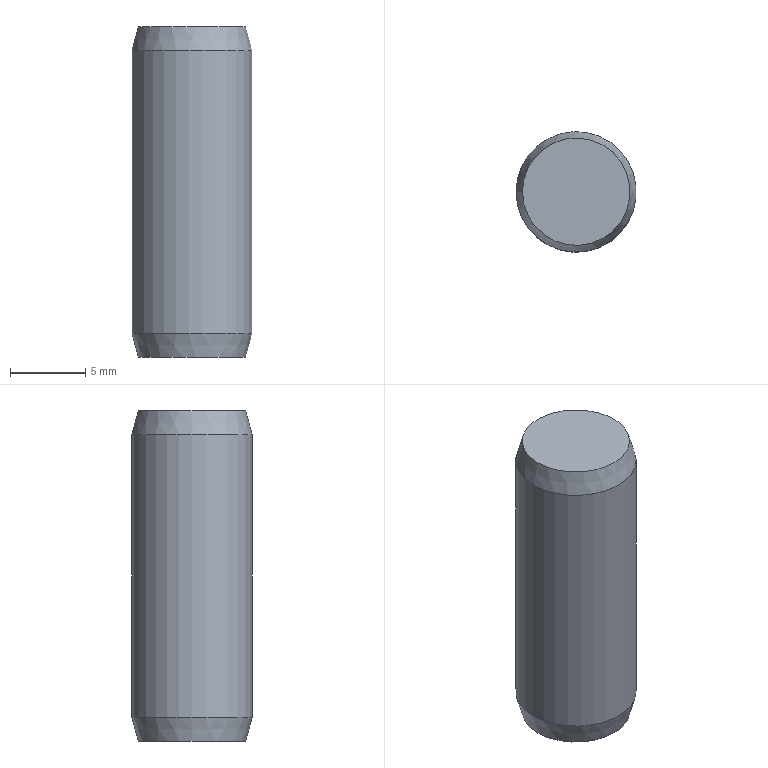Component | NX | GB-T119_1-2000_8X22 | 1 solid | 5 faces | box 8 x 8 x 22 mm | volume 1089 mm3 | plane 2 | cone 2 | cylinder 1 | commonest cylinder face diameters 8 x1
STEP:
#1=CARTESIAN_POINT('',(0.,0.,0.));
#2=DIRECTION('',(0.,0.,1.));
#3=DIRECTION('',(1.,0.,0.));
#4=AXIS2_PLACEMENT_3D('',#1,#2,#3);
#5=CARTESIAN_POINT('',(372.53,10.,-7.));
#6=VERTEX_POINT('',#5);
#7=CARTESIAN_POINT('',(376.101,10.,-7.));
#8=DIRECTION('',(0.,0.,-1.));
#9=DIRECTION('',(-1.,0.,0.));
#10=AXIS2_PLACEMENT_3D('',#7,#8,#9);
#11=CIRCLE('',#10,3.571);
#12=CARTESIAN_POINT('',(376.101,10.,-7.));
#13=DIRECTION('',(0.,0.,-1.));
#14=DIRECTION('',(-1.,0.,0.));
#15=AXIS2_PLACEMENT_3D('',#12,#13,#14);
#16=PLANE('',#15);
#17=CARTESIAN_POINT('',(0.,0.));
#18=DIRECTION('',(1.,0.));
#19=AXIS2_PLACEMENT_2D('',#17,#18);
#20=CIRCLE('',#19,3.571);
#21=(GEOMETRIC_REPRESENTATION_CONTEXT(2)PARAMETRIC_REPRESENTATION_CONTEXT()REPRESENTATION_CONTEXT('',''));
#22=DEFINITIONAL_REPRESENTATION('',(#20),#21);
#23=PCURVE('',#16,#22);
#24=CARTESIAN_POINT('',(376.101,10.,-7.));
#25=DIRECTION('',(0.,0.,1.));
#26=DIRECTION('',(1.,0.,0.));
#27=AXIS2_PLACEMENT_3D('',#24,#25,#26);
#28=CONICAL_SURFACE('',#27,3.571,0.2618);
#29=CARTESIAN_POINT('',(9.425,-0.));
#30=DIRECTION('',(-1.,0.));
#31=VECTOR('',#30,1.);
#32=LINE('',#29,#31);
#33=(GEOMETRIC_REPRESENTATION_CONTEXT(2)PARAMETRIC_REPRESENTATION_CONTEXT()REPRESENTATION_CONTEXT('',''));
#34=DEFINITIONAL_REPRESENTATION('',(#32),#33);
#35=PCURVE('',#28,#34);
#36=SURFACE_CURVE('',#11,(#23,#35),.PCURVE_S1.);
#37=EDGE_CURVE('',#6,#6,#36,.T.);
#38=ORIENTED_EDGE('',*,*,#37,.T.);
#39=EDGE_LOOP('',(#38));
#40=FACE_BOUND('',#39,.T.);
#41=ADVANCED_FACE('',(#40),#16,.T.);
#42=CARTESIAN_POINT('',(372.101,10.,-5.4));
#43=VERTEX_POINT('',#42);
#44=CARTESIAN_POINT('',(376.101,10.,-5.4));
#45=DIRECTION('',(0.,0.,-1.));
#46=DIRECTION('',(-1.,0.,0.));
#47=AXIS2_PLACEMENT_3D('',#44,#45,#46);
#48=CIRCLE('',#47,4.);
#49=CARTESIAN_POINT('',(9.425,1.6));
#50=DIRECTION('',(-1.,0.));
#51=VECTOR('',#50,1.);
#52=LINE('',#49,#51);
#53=(GEOMETRIC_REPRESENTATION_CONTEXT(2)PARAMETRIC_REPRESENTATION_CONTEXT()REPRESENTATION_CONTEXT('',''));
#54=DEFINITIONAL_REPRESENTATION('',(#52),#53);
#55=PCURVE('',#28,#54);
#56=CARTESIAN_POINT('',(376.101,10.,15.));
#57=DIRECTION('',(0.,0.,-1.));
#58=DIRECTION('',(-1.,0.,0.));
#59=AXIS2_PLACEMENT_3D('',#56,#57,#58);
#60=CYLINDRICAL_SURFACE('',#59,4.);
#61=CARTESIAN_POINT('',(0.,20.4));
#62=DIRECTION('',(1.,0.));
#63=VECTOR('',#62,1.);
#64=LINE('',#61,#63);
#65=(GEOMETRIC_REPRESENTATION_CONTEXT(2)PARAMETRIC_REPRESENTATION_CONTEXT()REPRESENTATION_CONTEXT('',''));
#66=DEFINITIONAL_REPRESENTATION('',(#64),#65);
#67=PCURVE('',#60,#66);
#68=SURFACE_CURVE('',#48,(#55,#67),.PCURVE_S1.);
#69=EDGE_CURVE('',#43,#43,#68,.T.);
#70=ORIENTED_EDGE('',*,*,#69,.T.);
#71=CARTESIAN_POINT('',(372.53,10.,-7.));
#72=CARTESIAN_POINT('',(372.101,10.,-5.4));
#73=B_SPLINE_CURVE_WITH_KNOTS('',1,(#71,#72),.UNSPECIFIED.,.F.,.F.,(2,2),(-0.,1.656),.PIECEWISE_BEZIER_KNOTS.);
#74=CARTESIAN_POINT('',(3.142,0.));
#75=DIRECTION('',(0.,1.));
#76=VECTOR('',#75,1.);
#77=LINE('',#74,#76);
#78=(GEOMETRIC_REPRESENTATION_CONTEXT(2)PARAMETRIC_REPRESENTATION_CONTEXT()REPRESENTATION_CONTEXT('',''));
#79=DEFINITIONAL_REPRESENTATION('',(#77),#78);
#80=PCURVE('',#28,#79);
#81=CARTESIAN_POINT('',(9.425,0.));
#82=DIRECTION('',(0.,1.));
#83=VECTOR('',#82,1.);
#84=LINE('',#81,#83);
#85=(GEOMETRIC_REPRESENTATION_CONTEXT(2)PARAMETRIC_REPRESENTATION_CONTEXT()REPRESENTATION_CONTEXT('',''));
#86=DEFINITIONAL_REPRESENTATION('',(#84),#85);
#87=PCURVE('',#28,#86);
#88=SEAM_CURVE('',#73,(#80,#87),.PCURVE_S1.);
#89=EDGE_CURVE('',#6,#43,#88,.T.);
#90=ORIENTED_EDGE('',*,*,#89,.F.);
#91=ORIENTED_EDGE('',*,*,#37,.F.);
#92=ORIENTED_EDGE('',*,*,#89,.T.);
#93=EDGE_LOOP('',(#70,#90,#91,#92));
#94=FACE_BOUND('',#93,.T.);
#95=ADVANCED_FACE('',(#94),#28,.T.);
#96=CARTESIAN_POINT('',(372.101,10.,13.4));
#97=VERTEX_POINT('',#96);
#98=CARTESIAN_POINT('',(376.101,10.,13.4));
#99=DIRECTION('',(0.,0.,-1.));
#100=DIRECTION('',(-1.,0.,0.));
#101=AXIS2_PLACEMENT_3D('',#98,#99,#100);
#102=CIRCLE('',#101,4.);
#103=CARTESIAN_POINT('',(0.,1.6));
#104=DIRECTION('',(1.,0.));
#105=VECTOR('',#104,1.);
#106=LINE('',#103,#105);
#107=(GEOMETRIC_REPRESENTATION_CONTEXT(2)PARAMETRIC_REPRESENTATION_CONTEXT()REPRESENTATION_CONTEXT('',''));
#108=DEFINITIONAL_REPRESENTATION('',(#106),#107);
#109=PCURVE('',#60,#108);
#110=CARTESIAN_POINT('',(376.101,10.,13.4));
#111=DIRECTION('',(0.,0.,-1.));
#112=DIRECTION('',(-1.,0.,0.));
#113=AXIS2_PLACEMENT_3D('',#110,#111,#112);
#114=CONICAL_SURFACE('',#113,4.,0.2618);
#115=CARTESIAN_POINT('',(0.,-0.));
#116=DIRECTION('',(1.,0.));
#117=VECTOR('',#116,1.);
#118=LINE('',#115,#117);
#119=(GEOMETRIC_REPRESENTATION_CONTEXT(2)PARAMETRIC_REPRESENTATION_CONTEXT()REPRESENTATION_CONTEXT('',''));
#120=DEFINITIONAL_REPRESENTATION('',(#118),#119);
#121=PCURVE('',#114,#120);
#122=SURFACE_CURVE('',#102,(#109,#121),.PCURVE_S1.);
#123=EDGE_CURVE('',#97,#97,#122,.T.);
#124=ORIENTED_EDGE('',*,*,#123,.T.);
#125=CARTESIAN_POINT('',(372.101,10.,13.4));
#126=CARTESIAN_POINT('',(372.101,10.,-5.4));
#127=B_SPLINE_CURVE_WITH_KNOTS('',1,(#125,#126),.UNSPECIFIED.,.F.,.F.,(2,2),(1.6,20.4),.PIECEWISE_BEZIER_KNOTS.);
#128=CARTESIAN_POINT('',(6.283,0.));
#129=DIRECTION('',(0.,1.));
#130=VECTOR('',#129,1.);
#131=LINE('',#128,#130);
#132=(GEOMETRIC_REPRESENTATION_CONTEXT(2)PARAMETRIC_REPRESENTATION_CONTEXT()REPRESENTATION_CONTEXT('',''));
#133=DEFINITIONAL_REPRESENTATION('',(#131),#132);
#134=PCURVE('',#60,#133);
#135=CARTESIAN_POINT('',(0.,0.));
#136=DIRECTION('',(0.,1.));
#137=VECTOR('',#136,1.);
#138=LINE('',#135,#137);
#139=(GEOMETRIC_REPRESENTATION_CONTEXT(2)PARAMETRIC_REPRESENTATION_CONTEXT()REPRESENTATION_CONTEXT('',''));
#140=DEFINITIONAL_REPRESENTATION('',(#138),#139);
#141=PCURVE('',#60,#140);
#142=SEAM_CURVE('',#127,(#134,#141),.PCURVE_S1.);
#143=EDGE_CURVE('',#97,#43,#142,.T.);
#144=ORIENTED_EDGE('',*,*,#143,.T.);
#145=ORIENTED_EDGE('',*,*,#69,.F.);
#146=ORIENTED_EDGE('',*,*,#143,.F.);
#147=EDGE_LOOP('',(#124,#144,#145,#146));
#148=FACE_BOUND('',#147,.T.);
#149=ADVANCED_FACE('',(#148),#60,.T.);
#150=CARTESIAN_POINT('',(372.53,10.,15.));
#151=VERTEX_POINT('',#150);
#152=CARTESIAN_POINT('',(376.101,10.,15.));
#153=DIRECTION('',(0.,0.,-1.));
#154=DIRECTION('',(-1.,0.,0.));
#155=AXIS2_PLACEMENT_3D('',#152,#153,#154);
#156=CIRCLE('',#155,3.571);
#157=CARTESIAN_POINT('',(0.,-1.6));
#158=DIRECTION('',(1.,0.));
#159=VECTOR('',#158,1.);
#160=LINE('',#157,#159);
#161=(GEOMETRIC_REPRESENTATION_CONTEXT(2)PARAMETRIC_REPRESENTATION_CONTEXT()REPRESENTATION_CONTEXT('',''));
#162=DEFINITIONAL_REPRESENTATION('',(#160),#161);
#163=PCURVE('',#114,#162);
#164=CARTESIAN_POINT('',(379.672,10.,15.));
#165=DIRECTION('',(0.,0.,1.));
#166=DIRECTION('',(1.,0.,0.));
#167=AXIS2_PLACEMENT_3D('',#164,#165,#166);
#168=PLANE('',#167);
#169=CARTESIAN_POINT('',(-7.143,0.));
#170=CARTESIAN_POINT('',(-7.143,6.186));
#171=CARTESIAN_POINT('',(-1.786,3.093));
#172=CARTESIAN_POINT('',(3.571,0.));
#173=CARTESIAN_POINT('',(-1.786,-3.093));
#174=CARTESIAN_POINT('',(-7.143,-6.186));
#175=CARTESIAN_POINT('',(-7.143,0.));
#176=(BOUNDED_CURVE()B_SPLINE_CURVE(2,(#169,#170,#171,#172,#173,#174,#175),.UNSPECIFIED.,.T.,.F.)B_SPLINE_CURVE_WITH_KNOTS((1,2,2,2,2,1),(-2.094,0.,2.094,4.189,6.283,8.378),.UNSPECIFIED.)CURVE()GEOMETRIC_REPRESENTATION_ITEM()RATIONAL_B_SPLINE_CURVE((1.,0.5,1.,0.5,1.,0.5,1.))REPRESENTATION_ITEM(''));
#177=(GEOMETRIC_REPRESENTATION_CONTEXT(2)PARAMETRIC_REPRESENTATION_CONTEXT()REPRESENTATION_CONTEXT('',''));
#178=DEFINITIONAL_REPRESENTATION('',(#176),#177);
#179=PCURVE('',#168,#178);
#180=SURFACE_CURVE('',#156,(#163,#179),.PCURVE_S1.);
#181=EDGE_CURVE('',#151,#151,#180,.T.);
#182=ORIENTED_EDGE('',*,*,#181,.T.);
#183=CARTESIAN_POINT('',(372.53,10.,15.));
#184=CARTESIAN_POINT('',(372.101,10.,13.4));
#185=B_SPLINE_CURVE_WITH_KNOTS('',1,(#183,#184),.UNSPECIFIED.,.F.,.F.,(2,2),(-1.656,-0.),.PIECEWISE_BEZIER_KNOTS.);
#186=CARTESIAN_POINT('',(6.283,0.));
#187=DIRECTION('',(0.,1.));
#188=VECTOR('',#187,1.);
#189=LINE('',#186,#188);
#190=(GEOMETRIC_REPRESENTATION_CONTEXT(2)PARAMETRIC_REPRESENTATION_CONTEXT()REPRESENTATION_CONTEXT('',''));
#191=DEFINITIONAL_REPRESENTATION('',(#189),#190);
#192=PCURVE('',#114,#191);
#193=CARTESIAN_POINT('',(0.,0.));
#194=DIRECTION('',(0.,1.));
#195=VECTOR('',#194,1.);
#196=LINE('',#193,#195);
#197=(GEOMETRIC_REPRESENTATION_CONTEXT(2)PARAMETRIC_REPRESENTATION_CONTEXT()REPRESENTATION_CONTEXT('',''));
#198=DEFINITIONAL_REPRESENTATION('',(#196),#197);
#199=PCURVE('',#114,#198);
#200=SEAM_CURVE('',#185,(#192,#199),.PCURVE_S1.);
#201=EDGE_CURVE('',#151,#97,#200,.T.);
#202=ORIENTED_EDGE('',*,*,#201,.T.);
#203=ORIENTED_EDGE('',*,*,#123,.F.);
#204=ORIENTED_EDGE('',*,*,#201,.F.);
#205=EDGE_LOOP('',(#182,#202,#203,#204));
#206=FACE_BOUND('',#205,.T.);
#207=ADVANCED_FACE('',(#206),#114,.T.);
#208=ORIENTED_EDGE('',*,*,#181,.F.);
#209=EDGE_LOOP('',(#208));
#210=FACE_BOUND('',#209,.T.);
#211=ADVANCED_FACE('',(#210),#168,.T.);
#212=CLOSED_SHELL('',(#41,#95,#149,#207,#211));
#213=MANIFOLD_SOLID_BREP('',#212);
#214=(LENGTH_UNIT()NAMED_UNIT(*)SI_UNIT(.MILLI.,.METRE.));
#215=UNCERTAINTY_MEASURE_WITH_UNIT(LENGTH_MEASURE(0.00001),#214,'','');
#216=(NAMED_UNIT(*)PLANE_ANGLE_UNIT()SI_UNIT($,.RADIAN.));
#217=(NAMED_UNIT(*)SI_UNIT($,.STERADIAN.)SOLID_ANGLE_UNIT());
#218=(GEOMETRIC_REPRESENTATION_CONTEXT(3)GLOBAL_UNCERTAINTY_ASSIGNED_CONTEXT((#215))GLOBAL_UNIT_ASSIGNED_CONTEXT((#214,#216,#217))REPRESENTATION_CONTEXT('',''));
#219=ADVANCED_BREP_SHAPE_REPRESENTATION('',(#4,#213),#218);